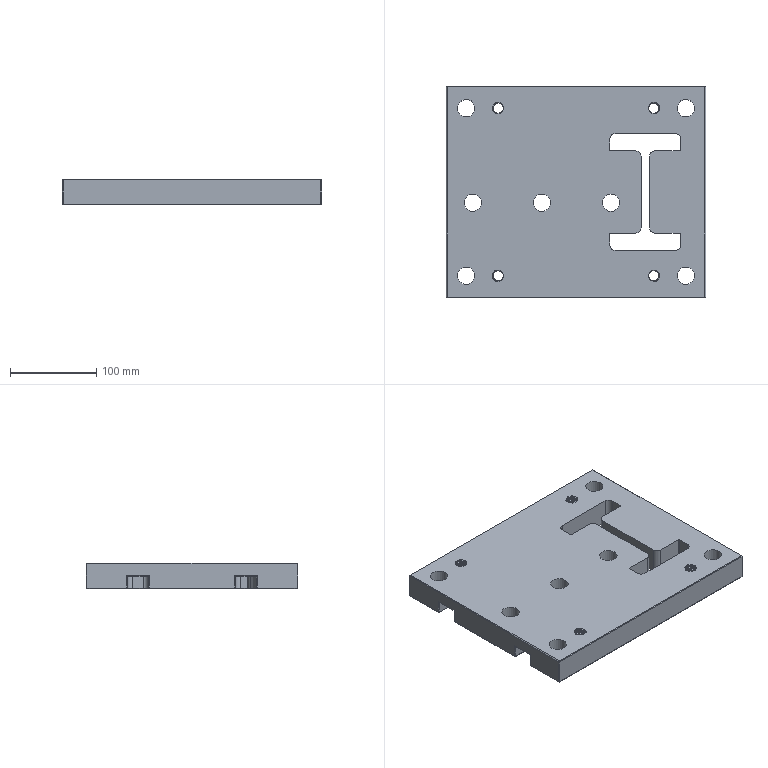Component | NX | STRIPPER | 1 solid | 115 faces | volume 1863542 mm3 | plane 66 | cylinder 34 | spline 8 | cone 7 | commonest cylinder face diameters 12 x8 20.015 x7 14 x4 12.015 x4 1.015 x4 11.985 x4 40 x2 20 x1